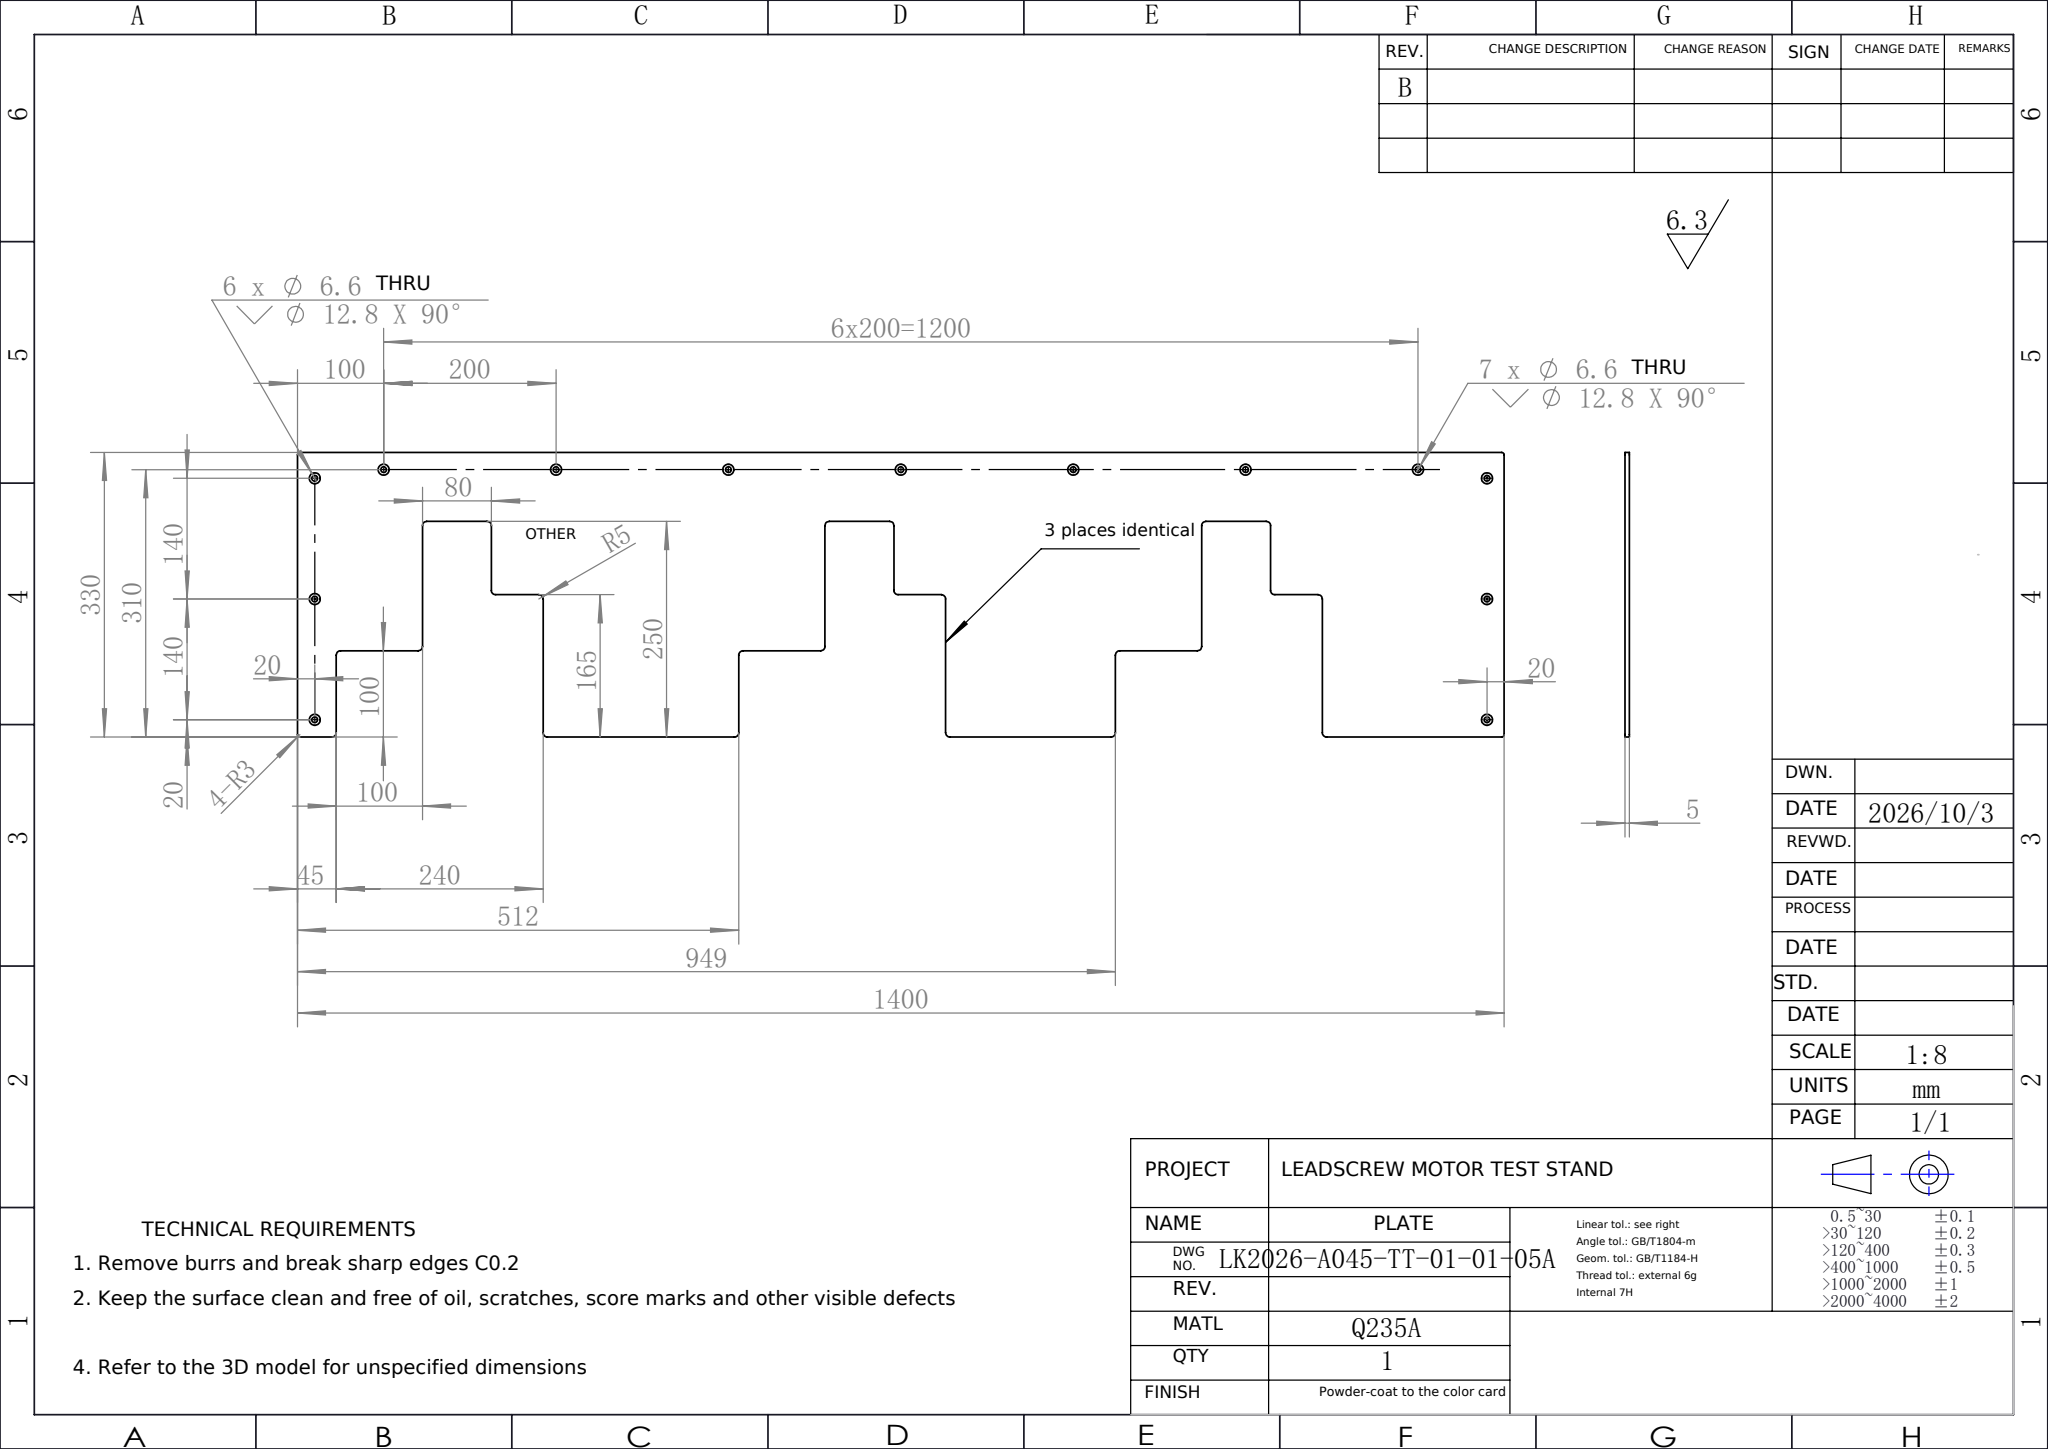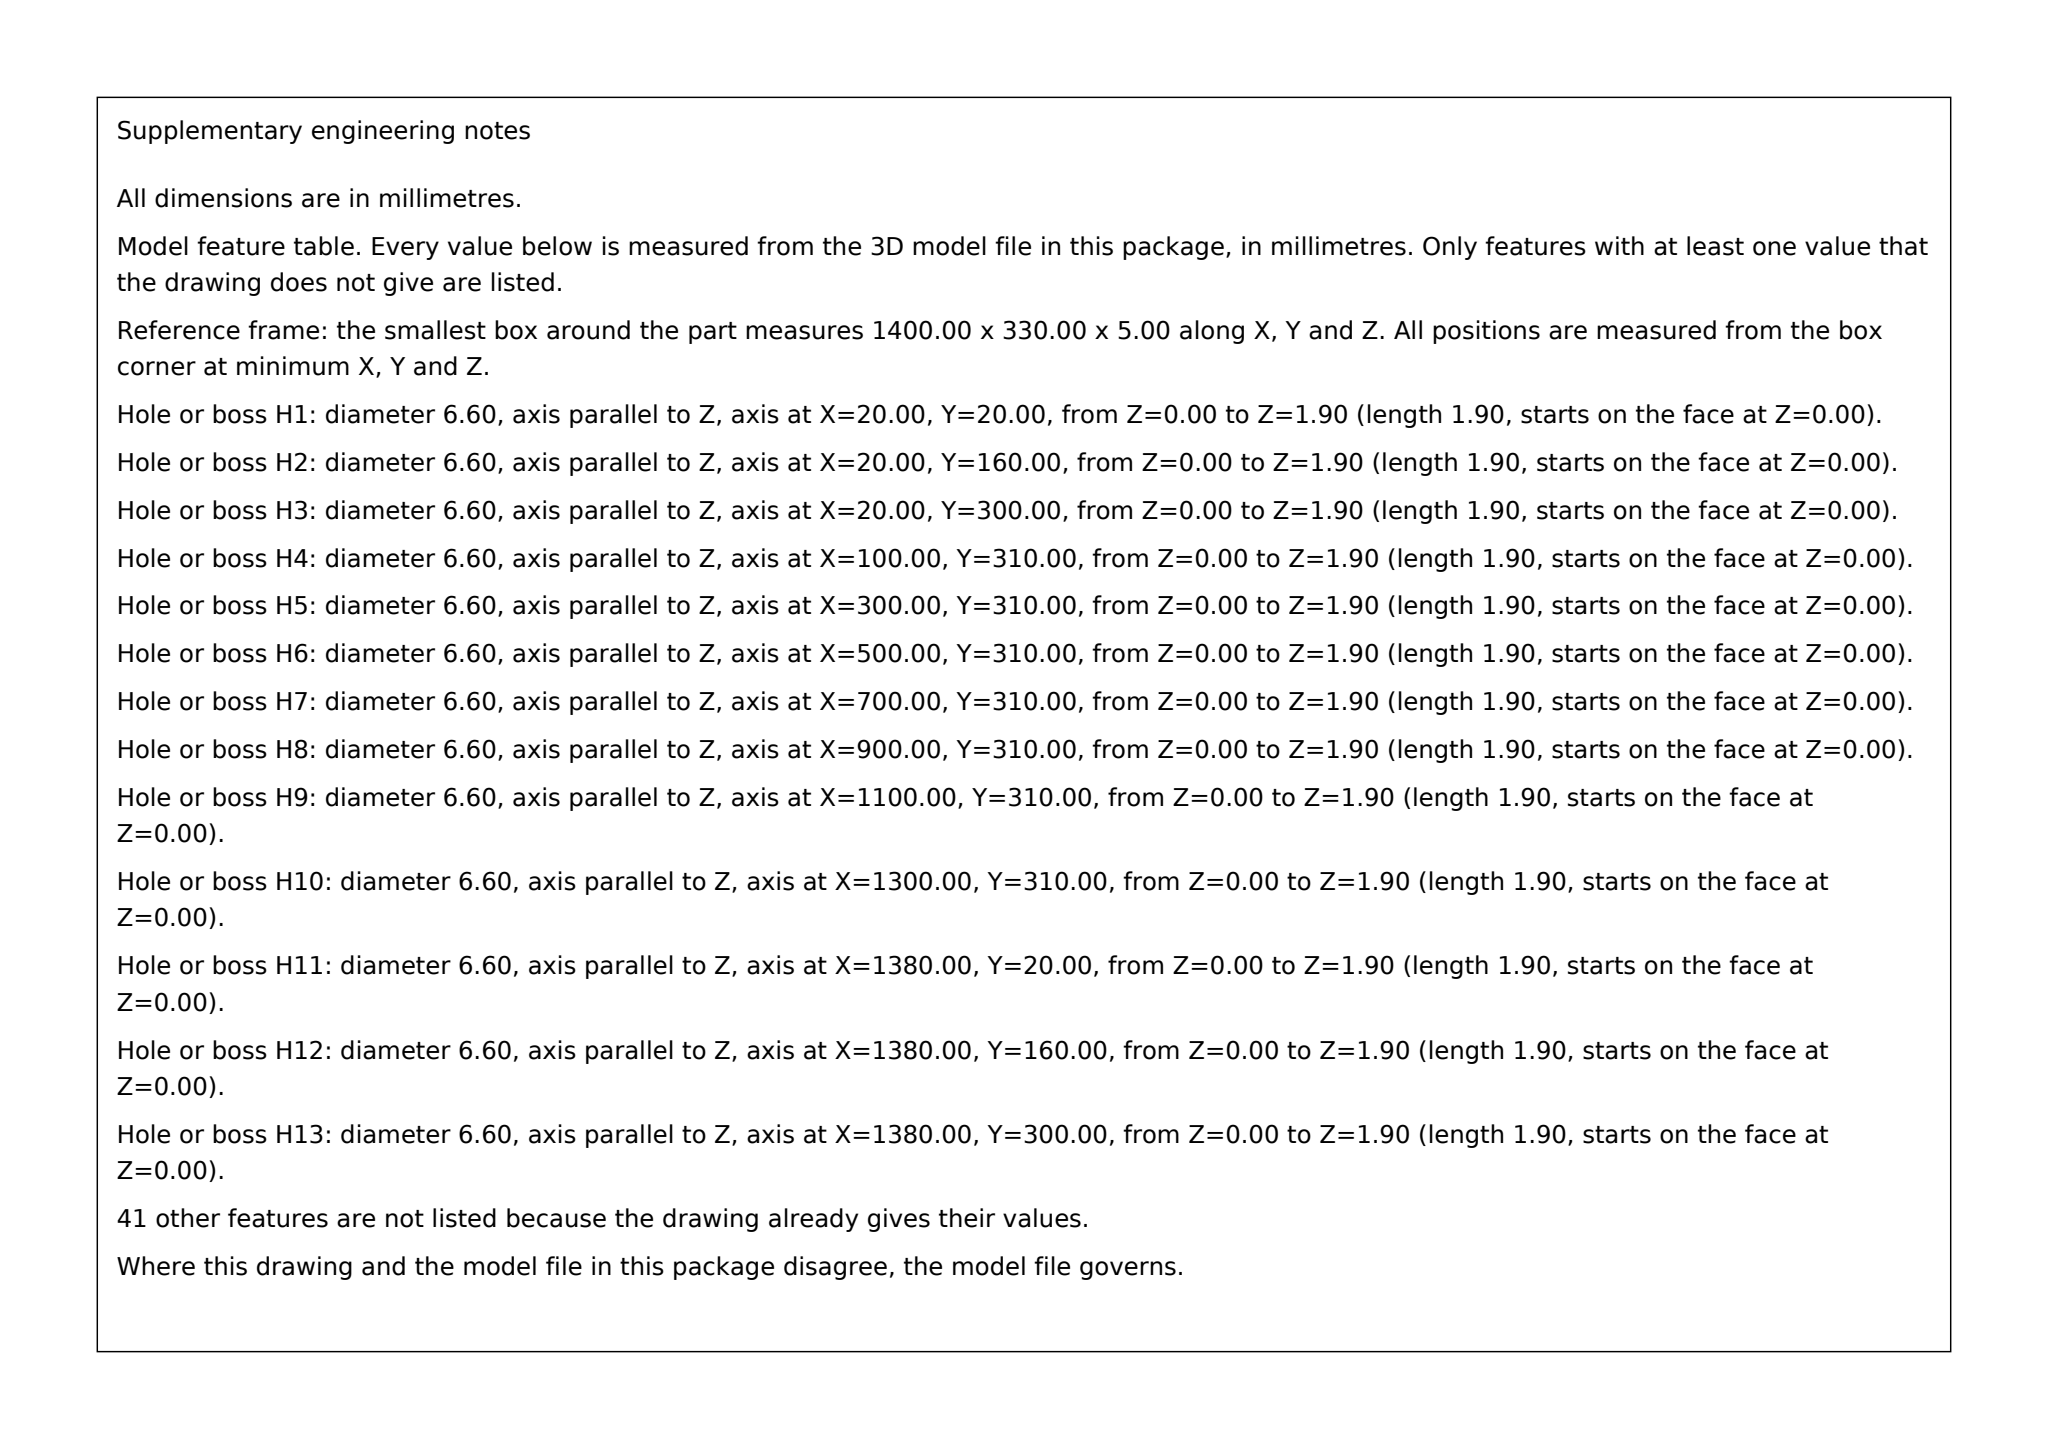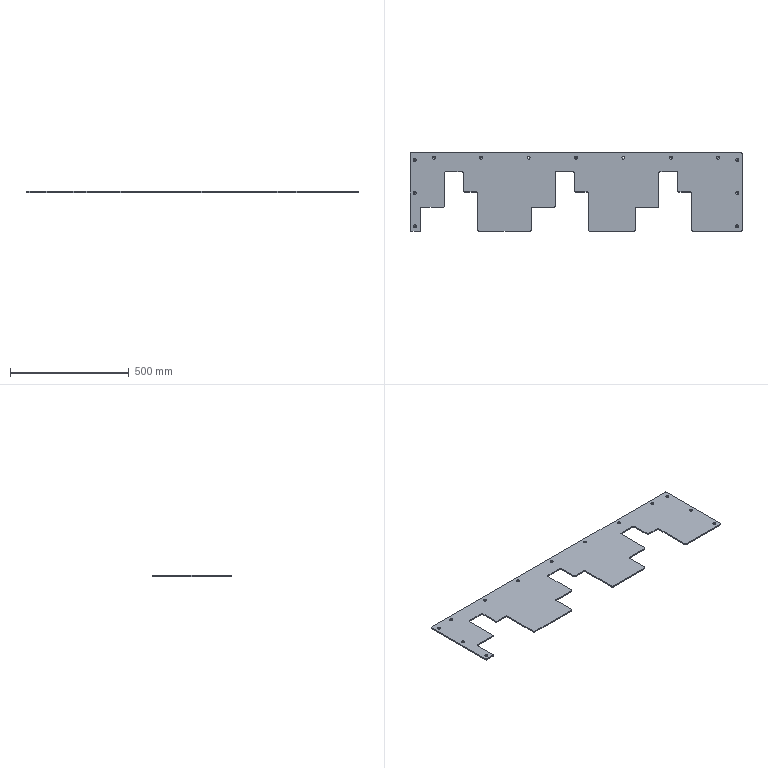Part | SolidWorks | mm | 1 solid | 110 faces | box 1400 x 330 x 5 mm | volume 1707537 mm3 | cylinder 54 | plane 30 | cone 26 | commonest cylinder face diameters 6.6 x26 10 x24 6 x4
build123d program:
from build123d import *

# Parameters (mm, degrees)
SKETCH1_W              = 1400
SKETCH1_H              = 330
BOSS_EXTRUDE1_DEPTH    = 5
FILLET2_R              = 3
LPATTERN1_COUNT        = 4
LPATTERN1_PITCH        = 200
LPATTERN2_COUNT        = 3
LPATTERN2_PITCH        = 140
CUT_EXTRUDE2_DEPTH     = 720.201
FILLET3_R              = 5
LPATTERN3_COUNT        = 2
LPATTERN3_PITCH        = 467
FILLET3_OF_LPATTERN3_R = 5
LPATTERN5_COUNT        = 2
LPATTERN5_PITCH        = 904
FILLET3_OF_LPATTERN5_R = 5


with BuildPart() as part:
    # Sketch1 → Boss-Extrude1 (new body)
    with BuildSketch(Plane.XY):
        Rectangle(SKETCH1_W, SKETCH1_H)
    extrude(amount=BOSS_EXTRUDE1_DEPTH)

    # Fillet2
    fillet2_edges = [part.edges().sort_by_distance(p)[0] for p in [
        (700, -165, 2.5),
        (-700, -165, 2.5),
        (-700, 165, 2.5),
        (700, 165, 2.5),
    ]]
    fillet(fillet2_edges, radius=FILLET2_R)

    # Sketch4 → Tapered Countersunk Hole 1 for M6 Hexalo (revolve, cut)
    with BuildSketch(Plane(origin=(0, 145, 5), x_dir=(0, -1, 0), z_dir=(1, 0, 0))):
        Polygon((0, 0), (0, 5), (3.3, 5), (3.3, 3.1), (6.4, 0), align=None)
    tapered_countersunk_hole_1_for_m6_hexalo = revolve(axis=Axis((0, 145, 11.35), (0, 0, -1)), mode=Mode.SUBTRACT)

    # LPattern1: Tapered Countersunk Hole 1 for M6 Hexalo ×4
    with Locations(*[(-i * LPATTERN1_PITCH, 0, 0) for i in range(1, LPATTERN1_COUNT)]):
        add(tapered_countersunk_hole_1_for_m6_hexalo, mode=Mode.SUBTRACT)

    # Mirror1 copy 1 sketch → Mirror1 copy 1 (revolve, cut)
    with BuildSketch(Plane(origin=(200, 145, 5), x_dir=(0, -1, 0), z_dir=(-1, 0, 0))):
        Polygon((0, 0), (0, -5), (3.3, -5), (3.3, -3.1), (6.4, 0), align=None)
    revolve(axis=Axis((200, 145, 11.35), (0, 0, 1)), mode=Mode.SUBTRACT)

    # Mirror1 copy 2 sketch → Mirror1 copy 2 (revolve, cut)
    with BuildSketch(Plane(origin=(400, 145, 5), x_dir=(0, -1, 0), z_dir=(-1, 0, 0))):
        Polygon((0, 0), (0, -5), (3.3, -5), (3.3, -3.1), (6.4, 0), align=None)
    revolve(axis=Axis((400, 145, 11.35), (0, 0, 1)), mode=Mode.SUBTRACT)

    # Mirror1 copy 3 sketch → Mirror1 copy 3 (revolve, cut)
    with BuildSketch(Plane(origin=(600, 145, 5), x_dir=(0, -1, 0), z_dir=(-1, 0, 0))):
        Polygon((0, 0), (0, -5), (3.3, -5), (3.3, -3.1), (6.4, 0), align=None)
    revolve(axis=Axis((600, 145, 11.35), (0, 0, 1)), mode=Mode.SUBTRACT)

    # Mirror1 copy 4 sketch → Mirror1 copy 4 (revolve, cut)
    with BuildSketch(Plane(origin=(0, 145, 5), x_dir=(0, -1, 0), z_dir=(-1, 0, 0))):
        Polygon((0, 0), (0, -5), (3.3, -5), (3.3, -3.1), (6.4, 0), align=None)
    revolve(axis=Axis((0, 145, 11.35), (0, 0, 1)), mode=Mode.SUBTRACT)

    # Sketch6 → Tapered Countersunk Hole 2 for M6 Hexalo (revolve, cut)
    with BuildSketch(Plane(origin=(-680, -145, 5), x_dir=(0, -1, 0), z_dir=(1, 0, 0))):
        Polygon((0, 0), (0, 5), (3.3, 5), (3.3, 3.1), (6.4, 0), align=None)
    tapered_countersunk_hole_2_for_m6_hexalo = revolve(axis=Axis((-680, -145, 11.35), (0, 0, -1)), mode=Mode.SUBTRACT)

    # LPattern2: Tapered Countersunk Hole 2 for M6 Hexalo ×3
    with Locations(*[(0, i * LPATTERN2_PITCH, 0) for i in range(1, LPATTERN2_COUNT)]):
        add(tapered_countersunk_hole_2_for_m6_hexalo, mode=Mode.SUBTRACT)

    # Mirror2: Tapered Countersunk Hole 2 for M6 Hexalo across plane
    add(tapered_countersunk_hole_2_for_m6_hexalo.mirror(Plane(origin=(0, 0, 0), x_dir=(0, 0, 1), z_dir=(1, 0, 0))), mode=Mode.SUBTRACT)

    # Mirror2 copy 1 sketch → Mirror2 copy 1 (revolve, cut)
    with BuildSketch(Plane(origin=(680, -5, 5), x_dir=(0, -1, 0), z_dir=(-1, 0, 0))):
        Polygon((0, 0), (0, -5), (3.3, -5), (3.3, -3.1), (6.4, 0), align=None)
    revolve(axis=Axis((680, -5, 11.35), (0, 0, 1)), mode=Mode.SUBTRACT)

    # Mirror2 copy 2 sketch → Mirror2 copy 2 (revolve, cut)
    with BuildSketch(Plane(origin=(680, 135, 5), x_dir=(0, -1, 0), z_dir=(-1, 0, 0))):
        Polygon((0, 0), (0, -5), (3.3, -5), (3.3, -3.1), (6.4, 0), align=None)
    revolve(axis=Axis((680, 135, 11.35), (0, 0, 1)), mode=Mode.SUBTRACT)

    # Sketch7 → Cut-Extrude2 (cut, through all)
    with BuildSketch(Plane.XY.offset(5)):
        Polygon((-555, -65), (-555, 85), (-475, 85), (-475, 0), (-415, 0), (-415, -165), (-655, -165), (-655, -65), align=None)
    cut_extrude2 = extrude(amount=-CUT_EXTRUDE2_DEPTH, mode=Mode.SUBTRACT)

    # Fillet3
    fillet3_edges = [part.edges().sort_by_distance(p)[0] for p in [
        (-655, -65, 2.5),
        (-555, -65, 2.5),
        (-555, 85, 2.5),
        (-475, 85, 2.5),
        (-475, 0, 2.5),
        (-415, 0, 2.5),
        (-415, -165, 2.5),
        (-655, -165, 2.5),
    ]]
    fillet(fillet3_edges, radius=FILLET3_R)

    # LPattern3: Cut-Extrude2 ×2
    with Locations(*[(i * LPATTERN3_PITCH, 0, 0) for i in range(1, LPATTERN3_COUNT)]):
        add(cut_extrude2, mode=Mode.SUBTRACT)

    # Fillet3 of LPattern3
    fillet3_of_lpattern3_edges = [part.edges().sort_by_distance(p)[0] for p in [
        (-188, -65, 2.5),
        (-88, -65, 2.5),
        (-88, 85, 2.5),
        (-8, 85, 2.5),
        (-8, 0, 2.5),
        (52, 0, 2.5),
        (52, -165, 2.5),
        (-188, -165, 2.5),
    ]]
    fillet(fillet3_of_lpattern3_edges, radius=FILLET3_OF_LPATTERN3_R)

    # LPattern5: Cut-Extrude2 ×2
    with Locations(*[(i * LPATTERN5_PITCH, 0, 0) for i in range(1, LPATTERN5_COUNT)]):
        add(cut_extrude2, mode=Mode.SUBTRACT)

    # Fillet3 of LPattern5
    fillet3_of_lpattern5_edges = [part.edges().sort_by_distance(p)[0] for p in [
        (249, -65, 2.5),
        (349, -65, 2.5),
        (349, 85, 2.5),
        (429, 85, 2.5),
        (429, 0, 2.5),
        (489, 0, 2.5),
        (489, -165, 2.5),
        (249, -165, 2.5),
    ]]
    fillet(fillet3_of_lpattern5_edges, radius=FILLET3_OF_LPATTERN5_R)


solid = part.part